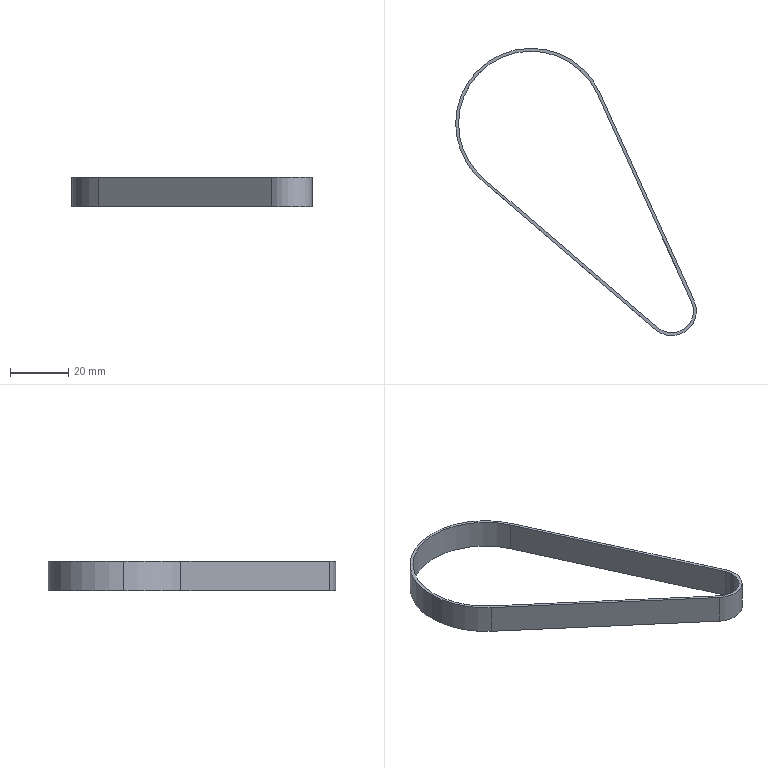Component | SolidWorks | Belt-1 | 1 solid | 12 faces | box 83.01 x 99.11 x 10 mm | volume 2706 mm3 | cylinder 6 | plane 6 | commonest cylinder face diameters 50 x2 52 x2 17 x1 15 x1
build123d program:
from build123d import *

# Parameters (mm, degrees)
EXTRUDE_THIN1_DEPTH = 10


with BuildPart() as part:
    # Sketch1 → Extrude-Thin1 (new body)
    with BuildSketch(Plane.XY):
        with BuildLine():
            Line((5.544, 24.865), (-54.35, -26.455))
            ThreePointArc((-54.35, -26.455), (-64.984, -26.797), (-67.622, -16.49))
            Line((-67.622, -16.49), (-35.053, 55.345))
            ThreePointArc((-35.053, 55.345), (4.237, 65.401), (5.544, 24.865))
        make_face()
        with BuildLine():
            Line((4.893, 25.624), (-55, -25.695))
            ThreePointArc((-55, -25.695), (-64.383, -25.998), (-66.711, -16.903))
            Line((-66.711, -16.903), (-34.143, 54.932))
            ThreePointArc((-34.143, 54.932), (3.636, 64.601), (4.893, 25.624))
        make_face(mode=Mode.SUBTRACT)
    extrude(amount=-EXTRUDE_THIN1_DEPTH)


solid = part.part

# Placed as in the assembly
solid = solid.moved(Location((-11.374, -44.609, -205), (-180, 0, 180)))
STEP:
#1=COLOUR_RGB('',0.7922,0.8196,0.9333);
#2=FILL_AREA_STYLE_COLOUR('',#1);
#3=FILL_AREA_STYLE('',(#2));
#4=SURFACE_STYLE_FILL_AREA(#3);
#5=SURFACE_SIDE_STYLE('',(#4));
#6=SURFACE_STYLE_USAGE(.BOTH.,#5);
#7=PRESENTATION_STYLE_ASSIGNMENT((#6));
#8=CARTESIAN_POINT('',(-0.9843,0.,-7.677));
#9=VERTEX_POINT('',#8);
#10=CARTESIAN_POINT('',(0.8964,0.4064,-7.677));
#11=VERTEX_POINT('',#10);
#12=CARTESIAN_POINT('',(0.,0.,-7.677));
#13=DIRECTION('',(0.,0.,-1.));
#14=DIRECTION('',(-1.,0.,0.));
#15=AXIS2_PLACEMENT_3D('',#12,#13,#14);
#16=CIRCLE('',#15,0.9843);
#17=EDGE_CURVE('',#9,#11,#16,.T.);
#18=ORIENTED_EDGE('',*,*,#17,.F.);
#19=CARTESIAN_POINT('',(-0.9843,0.,-8.071));
#20=VERTEX_POINT('',#19);
#21=CARTESIAN_POINT('',(-0.9843,0.,-7.677));
#22=DIRECTION('',(0.,0.,-1.));
#23=VECTOR('',#22,39.37);
#24=LINE('',#21,#23);
#25=EDGE_CURVE('',#9,#20,#24,.T.);
#26=ORIENTED_EDGE('',*,*,#25,.T.);
#27=CARTESIAN_POINT('',(0.8964,0.4064,-8.071));
#28=VERTEX_POINT('',#27);
#29=CARTESIAN_POINT('',(0.,0.,-8.071));
#30=DIRECTION('',(0.,0.,-1.));
#31=DIRECTION('',(-1.,0.,0.));
#32=AXIS2_PLACEMENT_3D('',#29,#30,#31);
#33=CIRCLE('',#32,0.9843);
#34=EDGE_CURVE('',#20,#28,#33,.T.);
#35=ORIENTED_EDGE('',*,*,#34,.T.);
#36=CARTESIAN_POINT('',(0.8964,0.4064,-7.677));
#37=DIRECTION('',(0.,0.,-1.));
#38=VECTOR('',#37,39.37);
#39=LINE('',#36,#38);
#40=EDGE_CURVE('',#11,#28,#39,.T.);
#41=ORIENTED_EDGE('',*,*,#40,.F.);
#42=EDGE_LOOP('',(#18,#26,#35,#41));
#43=FACE_OUTER_BOUND('',#42,.T.);
#44=CARTESIAN_POINT('',(0.,0.,-7.677));
#45=DIRECTION('',(0.,0.,-1.));
#46=DIRECTION('',(-1.,0.,0.));
#47=AXIS2_PLACEMENT_3D('',#44,#45,#46);
#48=CYLINDRICAL_SURFACE('',#47,0.9843);
#49=ADVANCED_FACE('',(#43),#48,.F.);
#50=CARTESIAN_POINT('',(-0.666,-0.7773,-7.677));
#51=VERTEX_POINT('',#50);
#52=CARTESIAN_POINT('',(-1.024,0.,-7.677));
#53=VERTEX_POINT('',#52);
#54=CARTESIAN_POINT('',(0.,0.,-7.677));
#55=DIRECTION('',(0.,0.,-1.));
#56=DIRECTION('',(-1.,0.,0.));
#57=AXIS2_PLACEMENT_3D('',#54,#55,#56);
#58=CIRCLE('',#57,1.024);
#59=EDGE_CURVE('',#51,#53,#58,.T.);
#60=ORIENTED_EDGE('',*,*,#59,.T.);
#61=CARTESIAN_POINT('',(-1.024,0.,-8.071));
#62=VERTEX_POINT('',#61);
#63=CARTESIAN_POINT('',(-1.024,0.,-7.677));
#64=DIRECTION('',(0.,0.,-1.));
#65=VECTOR('',#64,39.37);
#66=LINE('',#63,#65);
#67=EDGE_CURVE('',#53,#62,#66,.T.);
#68=ORIENTED_EDGE('',*,*,#67,.T.);
#69=CARTESIAN_POINT('',(-0.666,-0.7773,-8.071));
#70=VERTEX_POINT('',#69);
#71=CARTESIAN_POINT('',(0.,0.,-8.071));
#72=DIRECTION('',(0.,0.,-1.));
#73=DIRECTION('',(-1.,0.,0.));
#74=AXIS2_PLACEMENT_3D('',#71,#72,#73);
#75=CIRCLE('',#74,1.024);
#76=EDGE_CURVE('',#70,#62,#75,.T.);
#77=ORIENTED_EDGE('',*,*,#76,.F.);
#78=CARTESIAN_POINT('',(-0.666,-0.7773,-7.677));
#79=DIRECTION('',(0.,0.,-1.));
#80=VECTOR('',#79,39.37);
#81=LINE('',#78,#80);
#82=EDGE_CURVE('',#51,#70,#81,.T.);
#83=ORIENTED_EDGE('',*,*,#82,.F.);
#84=EDGE_LOOP('',(#60,#68,#77,#83));
#85=FACE_OUTER_BOUND('',#84,.T.);
#86=CARTESIAN_POINT('',(0.,0.,-7.677));
#87=DIRECTION('',(0.,0.,-1.));
#88=DIRECTION('',(-1.,0.,0.));
#89=AXIS2_PLACEMENT_3D('',#86,#87,#88);
#90=CYLINDRICAL_SURFACE('',#89,1.024);
#91=ADVANCED_FACE('',(#85),#90,.T.);
#92=CARTESIAN_POINT('',(2.214,-2.405,-8.071));
#93=VERTEX_POINT('',#92);
#94=CARTESIAN_POINT('',(1.692,-2.798,-8.071));
#95=VERTEX_POINT('',#94);
#96=CARTESIAN_POINT('',(1.91,-2.544,-8.071));
#97=DIRECTION('',(0.,0.,-1.));
#98=DIRECTION('',(-1.,0.,0.));
#99=AXIS2_PLACEMENT_3D('',#96,#97,#98);
#100=CIRCLE('',#99,0.3346);
#101=EDGE_CURVE('',#93,#95,#100,.T.);
#102=ORIENTED_EDGE('',*,*,#101,.F.);
#103=CARTESIAN_POINT('',(2.214,-2.405,-7.677));
#104=VERTEX_POINT('',#103);
#105=CARTESIAN_POINT('',(2.214,-2.405,-7.677));
#106=DIRECTION('',(0.,0.,-1.));
#107=VECTOR('',#106,39.37);
#108=LINE('',#105,#107);
#109=EDGE_CURVE('',#104,#93,#108,.T.);
#110=ORIENTED_EDGE('',*,*,#109,.F.);
#111=CARTESIAN_POINT('',(1.692,-2.798,-7.677));
#112=VERTEX_POINT('',#111);
#113=CARTESIAN_POINT('',(1.91,-2.544,-7.677));
#114=DIRECTION('',(0.,0.,-1.));
#115=DIRECTION('',(-1.,0.,0.));
#116=AXIS2_PLACEMENT_3D('',#113,#114,#115);
#117=CIRCLE('',#116,0.3346);
#118=EDGE_CURVE('',#104,#112,#117,.T.);
#119=ORIENTED_EDGE('',*,*,#118,.T.);
#120=CARTESIAN_POINT('',(1.692,-2.798,-7.677));
#121=DIRECTION('',(0.,0.,-1.));
#122=VECTOR('',#121,39.37);
#123=LINE('',#120,#122);
#124=EDGE_CURVE('',#112,#95,#123,.T.);
#125=ORIENTED_EDGE('',*,*,#124,.T.);
#126=EDGE_LOOP('',(#102,#110,#119,#125));
#127=FACE_OUTER_BOUND('',#126,.T.);
#128=CARTESIAN_POINT('',(1.91,-2.544,-7.677));
#129=DIRECTION('',(0.,0.,-1.));
#130=DIRECTION('',(-1.,0.,0.));
#131=AXIS2_PLACEMENT_3D('',#128,#129,#130);
#132=CYLINDRICAL_SURFACE('',#131,0.3346);
#133=ADVANCED_FACE('',(#127),#132,.T.);
#134=CARTESIAN_POINT('',(0.9323,0.4227,-8.071));
#135=VERTEX_POINT('',#134);
#136=CARTESIAN_POINT('',(2.214,-2.405,-8.071));
#137=DIRECTION('',(0.4129,-0.9108,0.));
#138=VECTOR('',#137,39.37);
#139=LINE('',#136,#138);
#140=EDGE_CURVE('',#135,#93,#139,.T.);
#141=ORIENTED_EDGE('',*,*,#140,.F.);
#142=CARTESIAN_POINT('',(0.9323,0.4227,-7.677));
#143=VERTEX_POINT('',#142);
#144=CARTESIAN_POINT('',(0.9323,0.4227,-7.677));
#145=DIRECTION('',(0.,0.,-1.));
#146=VECTOR('',#145,39.37);
#147=LINE('',#144,#146);
#148=EDGE_CURVE('',#143,#135,#147,.T.);
#149=ORIENTED_EDGE('',*,*,#148,.F.);
#150=CARTESIAN_POINT('',(2.214,-2.405,-7.677));
#151=DIRECTION('',(0.4129,-0.9108,0.));
#152=VECTOR('',#151,39.37);
#153=LINE('',#150,#152);
#154=EDGE_CURVE('',#143,#104,#153,.T.);
#155=ORIENTED_EDGE('',*,*,#154,.T.);
#156=ORIENTED_EDGE('',*,*,#109,.T.);
#157=EDGE_LOOP('',(#141,#149,#155,#156));
#158=FACE_OUTER_BOUND('',#157,.T.);
#159=CARTESIAN_POINT('',(2.214,-2.405,-7.677));
#160=DIRECTION('',(0.9108,0.4129,0.));
#161=DIRECTION('',(0.4129,-0.9108,0.));
#162=AXIS2_PLACEMENT_3D('',#159,#160,#161);
#163=PLANE('',#162);
#164=ADVANCED_FACE('',(#158),#163,.T.);
#165=ORIENTED_EDGE('',*,*,#67,.F.);
#166=CARTESIAN_POINT('',(0.,0.,-7.677));
#167=DIRECTION('',(0.,0.,-1.));
#168=DIRECTION('',(-1.,0.,0.));
#169=AXIS2_PLACEMENT_3D('',#166,#167,#168);
#170=CIRCLE('',#169,1.024);
#171=EDGE_CURVE('',#53,#143,#170,.T.);
#172=ORIENTED_EDGE('',*,*,#171,.T.);
#173=ORIENTED_EDGE('',*,*,#148,.T.);
#174=CARTESIAN_POINT('',(0.,0.,-8.071));
#175=DIRECTION('',(0.,0.,-1.));
#176=DIRECTION('',(-1.,0.,0.));
#177=AXIS2_PLACEMENT_3D('',#174,#175,#176);
#178=CIRCLE('',#177,1.024);
#179=EDGE_CURVE('',#62,#135,#178,.T.);
#180=ORIENTED_EDGE('',*,*,#179,.F.);
#181=EDGE_LOOP('',(#165,#172,#173,#180));
#182=FACE_OUTER_BOUND('',#181,.T.);
#183=CARTESIAN_POINT('',(0.,0.,-7.677));
#184=DIRECTION('',(0.,0.,-1.));
#185=DIRECTION('',(-1.,0.,0.));
#186=AXIS2_PLACEMENT_3D('',#183,#184,#185);
#187=CYLINDRICAL_SURFACE('',#186,1.024);
#188=ADVANCED_FACE('',(#182),#187,.T.);
#189=CARTESIAN_POINT('',(1.692,-2.798,-8.071));
#190=DIRECTION('',(-0.7594,0.6507,0.));
#191=VECTOR('',#190,39.37);
#192=LINE('',#189,#191);
#193=EDGE_CURVE('',#95,#70,#192,.T.);
#194=ORIENTED_EDGE('',*,*,#193,.F.);
#195=ORIENTED_EDGE('',*,*,#124,.F.);
#196=CARTESIAN_POINT('',(1.692,-2.798,-7.677));
#197=DIRECTION('',(-0.7594,0.6507,0.));
#198=VECTOR('',#197,39.37);
#199=LINE('',#196,#198);
#200=EDGE_CURVE('',#112,#51,#199,.T.);
#201=ORIENTED_EDGE('',*,*,#200,.T.);
#202=ORIENTED_EDGE('',*,*,#82,.T.);
#203=EDGE_LOOP('',(#194,#195,#201,#202));
#204=FACE_OUTER_BOUND('',#203,.T.);
#205=CARTESIAN_POINT('',(1.692,-2.798,-7.677));
#206=DIRECTION('',(-0.6507,-0.7594,0.));
#207=DIRECTION('',(-0.7594,0.6507,0.));
#208=AXIS2_PLACEMENT_3D('',#205,#206,#207);
#209=PLANE('',#208);
#210=ADVANCED_FACE('',(#204),#209,.T.);
#211=CARTESIAN_POINT('',(2.179,-2.422,-7.677));
#212=VERTEX_POINT('',#211);
#213=CARTESIAN_POINT('',(2.179,-2.422,-7.677));
#214=DIRECTION('',(0.4129,-0.9108,0.));
#215=VECTOR('',#214,39.37);
#216=LINE('',#213,#215);
#217=EDGE_CURVE('',#11,#212,#216,.T.);
#218=ORIENTED_EDGE('',*,*,#217,.T.);
#219=CARTESIAN_POINT('',(1.718,-2.768,-7.677));
#220=VERTEX_POINT('',#219);
#221=CARTESIAN_POINT('',(1.91,-2.544,-7.677));
#222=DIRECTION('',(0.,0.,-1.));
#223=DIRECTION('',(-1.,0.,0.));
#224=AXIS2_PLACEMENT_3D('',#221,#222,#223);
#225=CIRCLE('',#224,0.2953);
#226=EDGE_CURVE('',#212,#220,#225,.T.);
#227=ORIENTED_EDGE('',*,*,#226,.T.);
#228=CARTESIAN_POINT('',(-0.6404,-0.7474,-7.677));
#229=VERTEX_POINT('',#228);
#230=CARTESIAN_POINT('',(1.718,-2.768,-7.677));
#231=DIRECTION('',(-0.7594,0.6507,0.));
#232=VECTOR('',#231,39.37);
#233=LINE('',#230,#232);
#234=EDGE_CURVE('',#220,#229,#233,.T.);
#235=ORIENTED_EDGE('',*,*,#234,.T.);
#236=CARTESIAN_POINT('',(0.,0.,-7.677));
#237=DIRECTION('',(0.,0.,-1.));
#238=DIRECTION('',(-1.,0.,0.));
#239=AXIS2_PLACEMENT_3D('',#236,#237,#238);
#240=CIRCLE('',#239,0.9843);
#241=EDGE_CURVE('',#229,#9,#240,.T.);
#242=ORIENTED_EDGE('',*,*,#241,.T.);
#243=ORIENTED_EDGE('',*,*,#17,.T.);
#244=EDGE_LOOP('',(#218,#227,#235,#242,#243));
#245=FACE_BOUND('',#244,.T.);
#246=ORIENTED_EDGE('',*,*,#118,.F.);
#247=ORIENTED_EDGE('',*,*,#154,.F.);
#248=ORIENTED_EDGE('',*,*,#171,.F.);
#249=ORIENTED_EDGE('',*,*,#59,.F.);
#250=ORIENTED_EDGE('',*,*,#200,.F.);
#251=EDGE_LOOP('',(#246,#247,#248,#249,#250));
#252=FACE_OUTER_BOUND('',#251,.T.);
#253=CARTESIAN_POINT('',(1.91,-2.544,-7.677));
#254=DIRECTION('',(0.,0.,-1.));
#255=DIRECTION('',(-1.,0.,0.));
#256=AXIS2_PLACEMENT_3D('',#253,#254,#255);
#257=PLANE('',#256);
#258=ADVANCED_FACE('',(#245,#252),#257,.F.);
#259=CARTESIAN_POINT('',(2.179,-2.422,-8.071));
#260=VERTEX_POINT('',#259);
#261=CARTESIAN_POINT('',(1.718,-2.768,-8.071));
#262=VERTEX_POINT('',#261);
#263=CARTESIAN_POINT('',(1.91,-2.544,-8.071));
#264=DIRECTION('',(0.,0.,-1.));
#265=DIRECTION('',(-1.,0.,0.));
#266=AXIS2_PLACEMENT_3D('',#263,#264,#265);
#267=CIRCLE('',#266,0.2953);
#268=EDGE_CURVE('',#260,#262,#267,.T.);
#269=ORIENTED_EDGE('',*,*,#268,.F.);
#270=CARTESIAN_POINT('',(2.179,-2.422,-8.071));
#271=DIRECTION('',(0.4129,-0.9108,0.));
#272=VECTOR('',#271,39.37);
#273=LINE('',#270,#272);
#274=EDGE_CURVE('',#28,#260,#273,.T.);
#275=ORIENTED_EDGE('',*,*,#274,.F.);
#276=ORIENTED_EDGE('',*,*,#34,.F.);
#277=CARTESIAN_POINT('',(-0.6404,-0.7474,-8.071));
#278=VERTEX_POINT('',#277);
#279=CARTESIAN_POINT('',(0.,0.,-8.071));
#280=DIRECTION('',(0.,0.,-1.));
#281=DIRECTION('',(-1.,0.,0.));
#282=AXIS2_PLACEMENT_3D('',#279,#280,#281);
#283=CIRCLE('',#282,0.9843);
#284=EDGE_CURVE('',#278,#20,#283,.T.);
#285=ORIENTED_EDGE('',*,*,#284,.F.);
#286=CARTESIAN_POINT('',(1.718,-2.768,-8.071));
#287=DIRECTION('',(-0.7594,0.6507,0.));
#288=VECTOR('',#287,39.37);
#289=LINE('',#286,#288);
#290=EDGE_CURVE('',#262,#278,#289,.T.);
#291=ORIENTED_EDGE('',*,*,#290,.F.);
#292=EDGE_LOOP('',(#269,#275,#276,#285,#291));
#293=FACE_BOUND('',#292,.T.);
#294=ORIENTED_EDGE('',*,*,#101,.T.);
#295=ORIENTED_EDGE('',*,*,#193,.T.);
#296=ORIENTED_EDGE('',*,*,#76,.T.);
#297=ORIENTED_EDGE('',*,*,#179,.T.);
#298=ORIENTED_EDGE('',*,*,#140,.T.);
#299=EDGE_LOOP('',(#294,#295,#296,#297,#298));
#300=FACE_OUTER_BOUND('',#299,.T.);
#301=CARTESIAN_POINT('',(1.91,-2.544,-8.071));
#302=DIRECTION('',(0.,0.,-1.));
#303=DIRECTION('',(-1.,0.,0.));
#304=AXIS2_PLACEMENT_3D('',#301,#302,#303);
#305=PLANE('',#304);
#306=ADVANCED_FACE('',(#293,#300),#305,.T.);
#307=ORIENTED_EDGE('',*,*,#268,.T.);
#308=CARTESIAN_POINT('',(1.718,-2.768,-7.677));
#309=DIRECTION('',(0.,0.,-1.));
#310=VECTOR('',#309,39.37);
#311=LINE('',#308,#310);
#312=EDGE_CURVE('',#220,#262,#311,.T.);
#313=ORIENTED_EDGE('',*,*,#312,.F.);
#314=ORIENTED_EDGE('',*,*,#226,.F.);
#315=CARTESIAN_POINT('',(2.179,-2.422,-7.677));
#316=DIRECTION('',(0.,0.,-1.));
#317=VECTOR('',#316,39.37);
#318=LINE('',#315,#317);
#319=EDGE_CURVE('',#212,#260,#318,.T.);
#320=ORIENTED_EDGE('',*,*,#319,.T.);
#321=EDGE_LOOP('',(#307,#313,#314,#320));
#322=FACE_OUTER_BOUND('',#321,.T.);
#323=CARTESIAN_POINT('',(1.91,-2.544,-7.677));
#324=DIRECTION('',(0.,0.,-1.));
#325=DIRECTION('',(-1.,0.,0.));
#326=AXIS2_PLACEMENT_3D('',#323,#324,#325);
#327=CYLINDRICAL_SURFACE('',#326,0.2953);
#328=ADVANCED_FACE('',(#322),#327,.F.);
#329=ORIENTED_EDGE('',*,*,#274,.T.);
#330=ORIENTED_EDGE('',*,*,#319,.F.);
#331=ORIENTED_EDGE('',*,*,#217,.F.);
#332=ORIENTED_EDGE('',*,*,#40,.T.);
#333=EDGE_LOOP('',(#329,#330,#331,#332));
#334=FACE_OUTER_BOUND('',#333,.T.);
#335=CARTESIAN_POINT('',(2.179,-2.422,-7.677));
#336=DIRECTION('',(0.9108,0.4129,0.));
#337=DIRECTION('',(0.4129,-0.9108,0.));
#338=AXIS2_PLACEMENT_3D('',#335,#336,#337);
#339=PLANE('',#338);
#340=ADVANCED_FACE('',(#334),#339,.F.);
#341=ORIENTED_EDGE('',*,*,#25,.F.);
#342=ORIENTED_EDGE('',*,*,#241,.F.);
#343=CARTESIAN_POINT('',(-0.6404,-0.7474,-7.677));
#344=DIRECTION('',(0.,0.,-1.));
#345=VECTOR('',#344,39.37);
#346=LINE('',#343,#345);
#347=EDGE_CURVE('',#229,#278,#346,.T.);
#348=ORIENTED_EDGE('',*,*,#347,.T.);
#349=ORIENTED_EDGE('',*,*,#284,.T.);
#350=EDGE_LOOP('',(#341,#342,#348,#349));
#351=FACE_OUTER_BOUND('',#350,.T.);
#352=CARTESIAN_POINT('',(0.,0.,-7.677));
#353=DIRECTION('',(0.,0.,-1.));
#354=DIRECTION('',(-1.,0.,0.));
#355=AXIS2_PLACEMENT_3D('',#352,#353,#354);
#356=CYLINDRICAL_SURFACE('',#355,0.9843);
#357=ADVANCED_FACE('',(#351),#356,.F.);
#358=ORIENTED_EDGE('',*,*,#290,.T.);
#359=ORIENTED_EDGE('',*,*,#347,.F.);
#360=ORIENTED_EDGE('',*,*,#234,.F.);
#361=ORIENTED_EDGE('',*,*,#312,.T.);
#362=EDGE_LOOP('',(#358,#359,#360,#361));
#363=FACE_OUTER_BOUND('',#362,.T.);
#364=CARTESIAN_POINT('',(1.718,-2.768,-7.677));
#365=DIRECTION('',(-0.6507,-0.7594,0.));
#366=DIRECTION('',(-0.7594,0.6507,0.));
#367=AXIS2_PLACEMENT_3D('',#364,#365,#366);
#368=PLANE('',#367);
#369=ADVANCED_FACE('',(#363),#368,.F.);
#370=CLOSED_SHELL('',(#49,#91,#133,#164,#188,#210,#258,#306,#328,#340,#357,#369));
#371=MANIFOLD_SOLID_BREP('',#370);
#372=STYLED_ITEM('',(#7),#371);
#373=(LENGTH_UNIT()NAMED_UNIT(*)SI_UNIT($,.METRE.));
#374=LENGTH_MEASURE_WITH_UNIT(LENGTH_MEASURE(0.0254),#373);
#375=DIMENSIONAL_EXPONENTS(1.,0.,0.,0.,0.,0.,0.);
#376=(CONVERSION_BASED_UNIT('',#374)LENGTH_UNIT()NAMED_UNIT(#375));
#377=UNCERTAINTY_MEASURE_WITH_UNIT(LENGTH_MEASURE(0.00001),#376,'','');
#378=(NAMED_UNIT(*)PLANE_ANGLE_UNIT()SI_UNIT($,.RADIAN.));
#379=(NAMED_UNIT(*)SI_UNIT($,.STERADIAN.)SOLID_ANGLE_UNIT());
#380=(GEOMETRIC_REPRESENTATION_CONTEXT(3)GLOBAL_UNCERTAINTY_ASSIGNED_CONTEXT((#377))GLOBAL_UNIT_ASSIGNED_CONTEXT((#376,#378,#379))REPRESENTATION_CONTEXT('',''));
#381=MECHANICAL_DESIGN_GEOMETRIC_PRESENTATION_REPRESENTATION('',(#372),#380);
#382=PRESENTATION_LAYER_ASSIGNMENT('','',(#372));
#383=CARTESIAN_POINT('',(0.,0.,0.));
#384=DIRECTION('',(0.,0.,1.));
#385=DIRECTION('',(1.,0.,0.));
#386=AXIS2_PLACEMENT_3D('',#383,#384,#385);
#387=(LENGTH_UNIT()NAMED_UNIT(*)SI_UNIT($,.METRE.));
#388=LENGTH_MEASURE_WITH_UNIT(LENGTH_MEASURE(0.0254),#387);
#389=DIMENSIONAL_EXPONENTS(1.,0.,0.,0.,0.,0.,0.);
#390=(CONVERSION_BASED_UNIT('',#388)LENGTH_UNIT()NAMED_UNIT(#389));
#391=UNCERTAINTY_MEASURE_WITH_UNIT(LENGTH_MEASURE(0.00001),#390,'','');
#392=(NAMED_UNIT(*)PLANE_ANGLE_UNIT()SI_UNIT($,.RADIAN.));
#393=(NAMED_UNIT(*)SI_UNIT($,.STERADIAN.)SOLID_ANGLE_UNIT());
#394=(GEOMETRIC_REPRESENTATION_CONTEXT(3)GLOBAL_UNCERTAINTY_ASSIGNED_CONTEXT((#391))GLOBAL_UNIT_ASSIGNED_CONTEXT((#390,#392,#393))REPRESENTATION_CONTEXT('',''));
#395=ADVANCED_BREP_SHAPE_REPRESENTATION('',(#371,#386),#394);